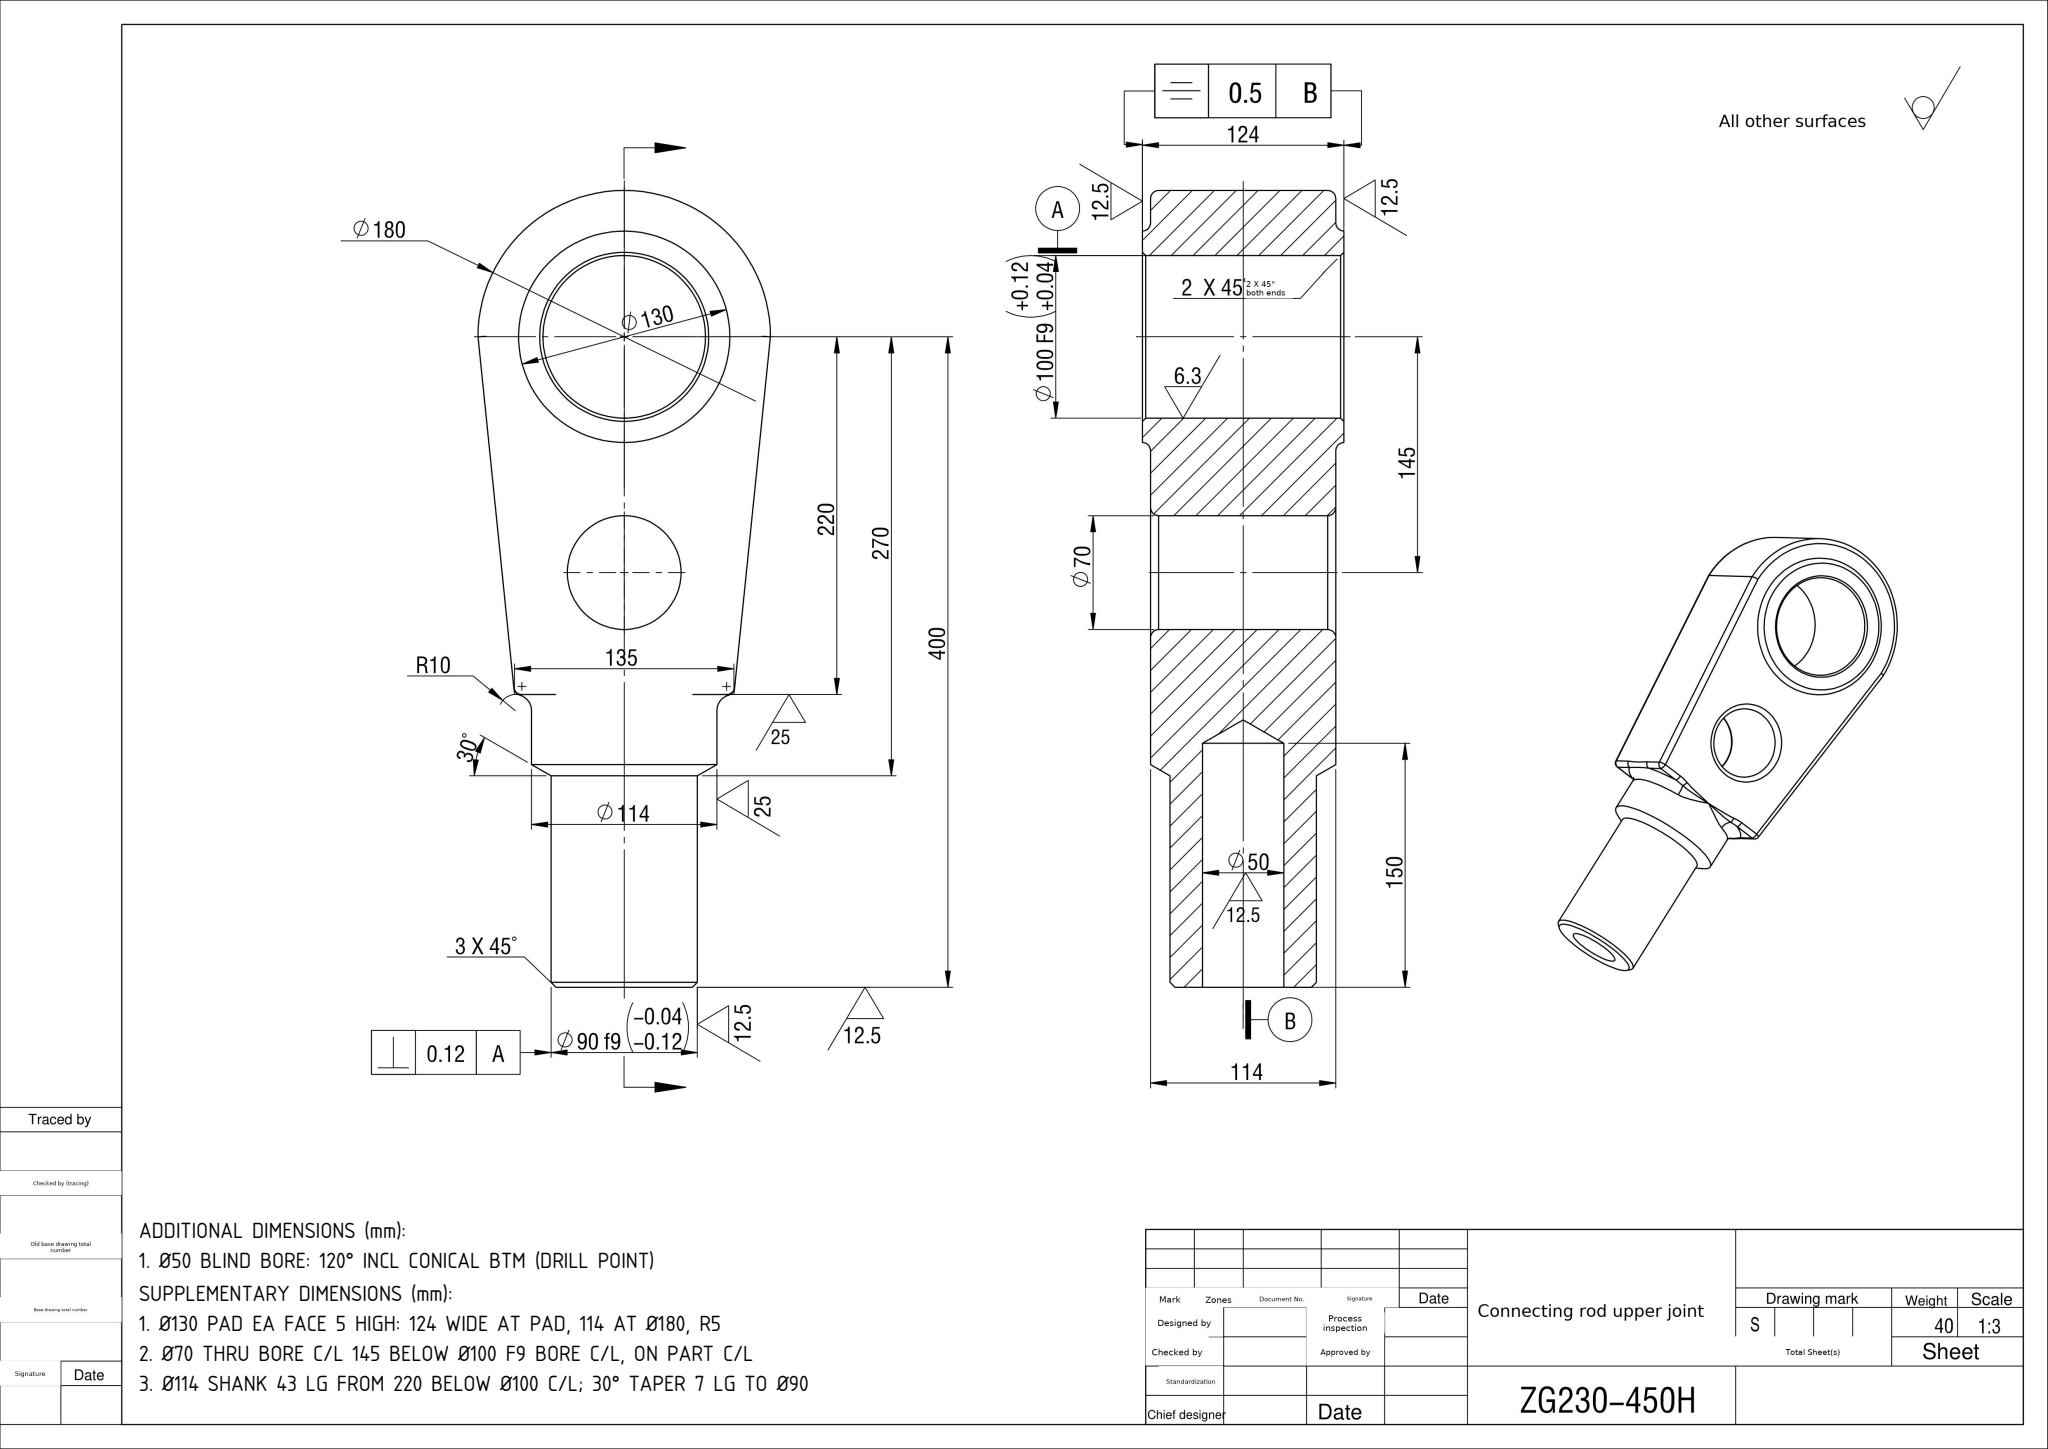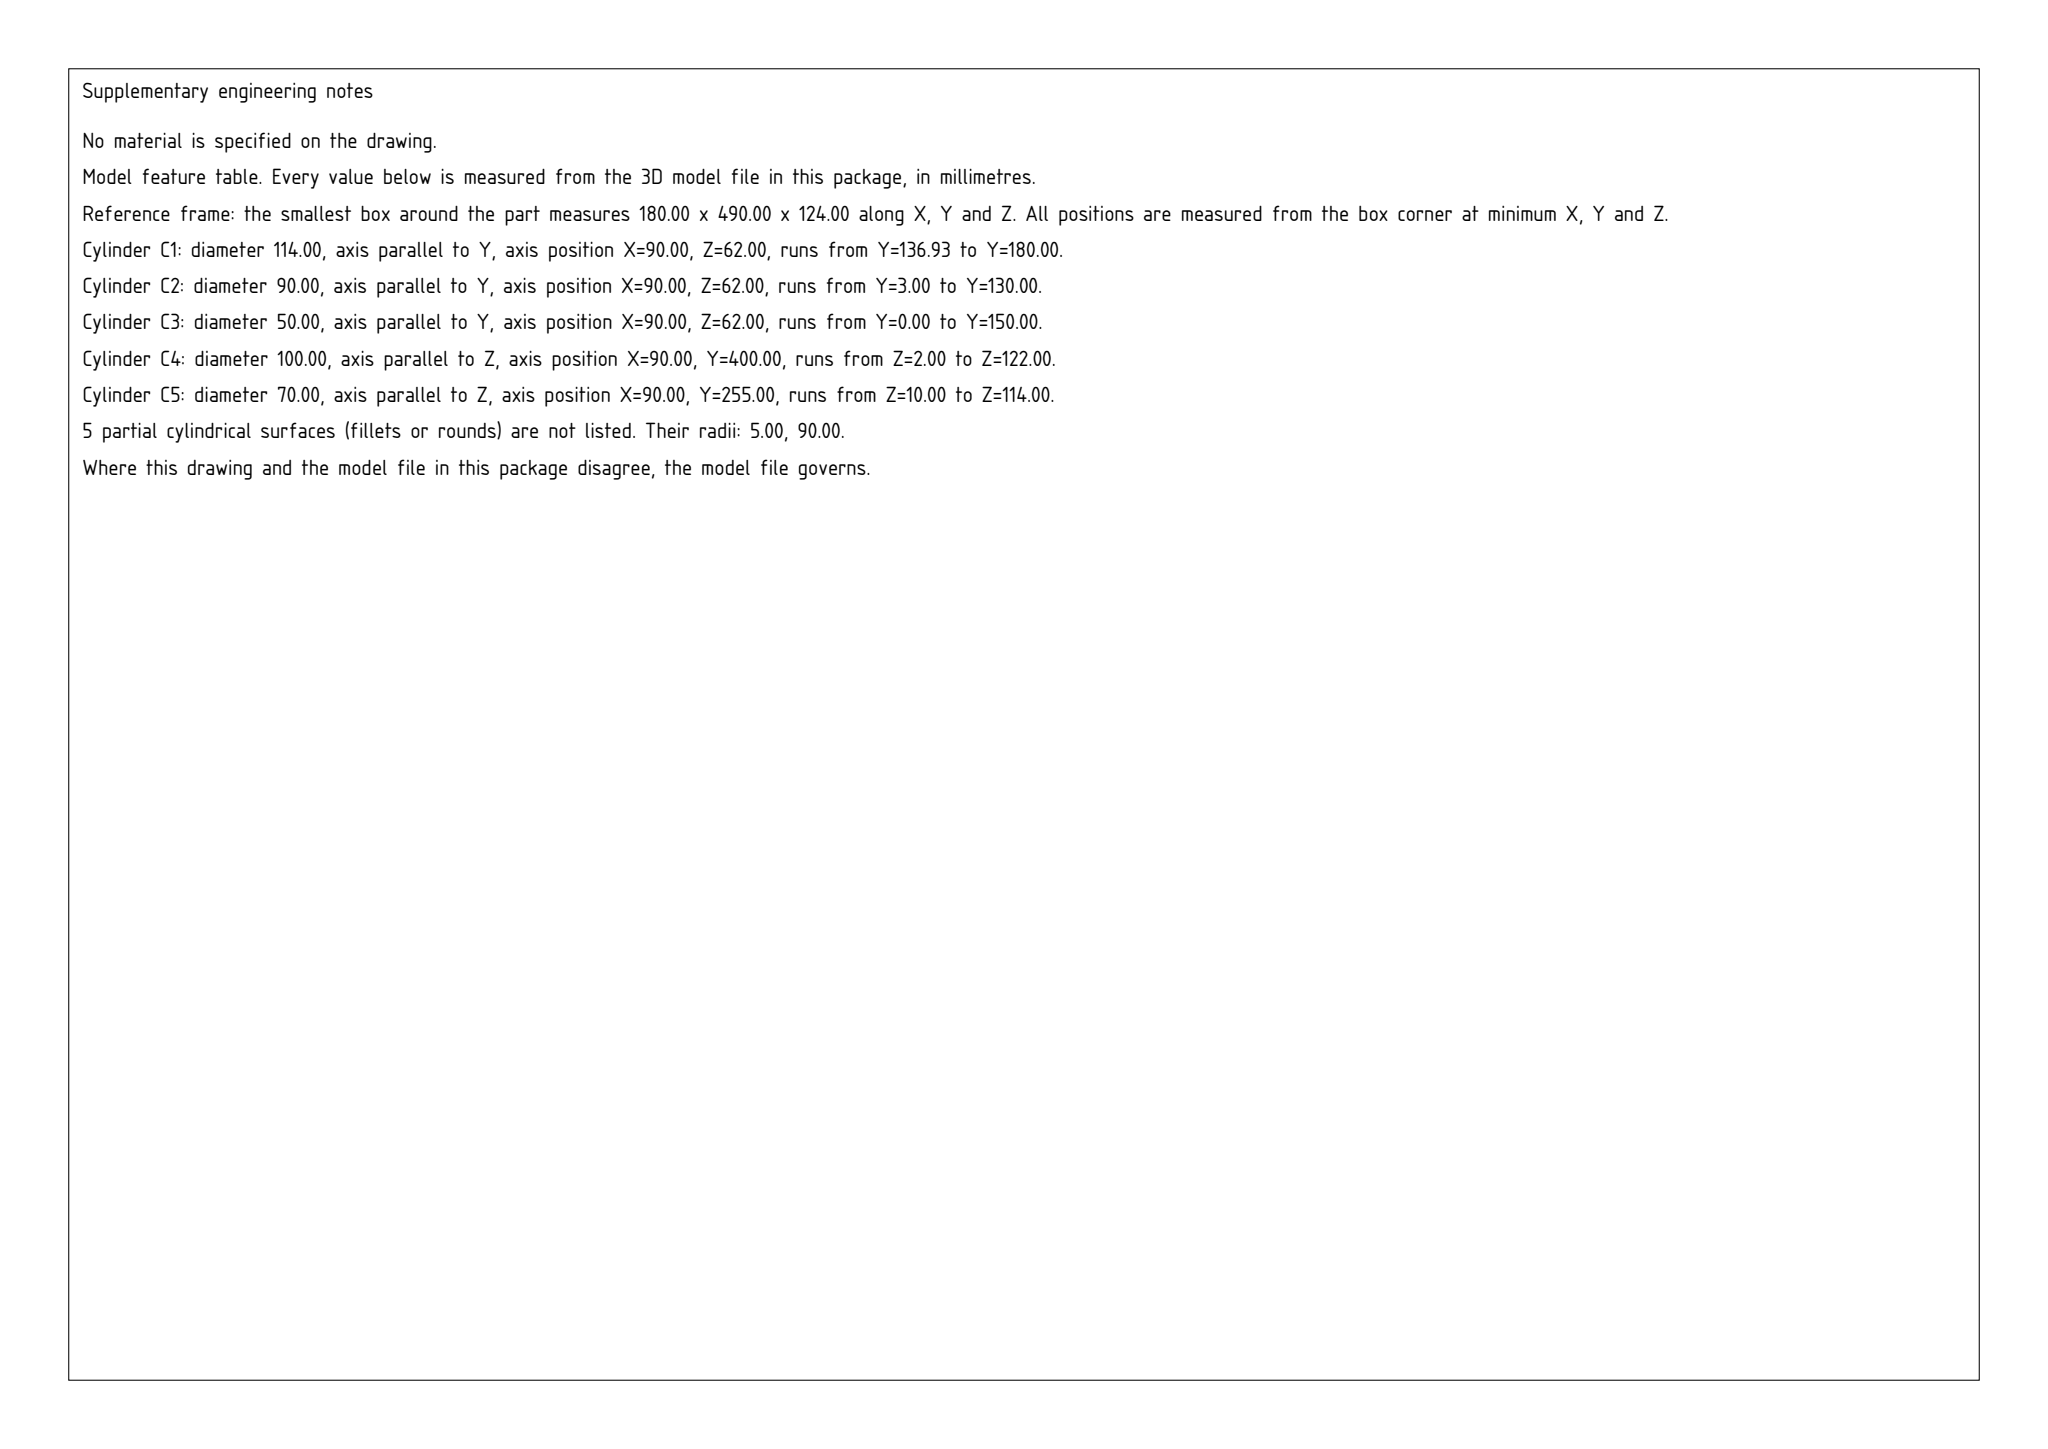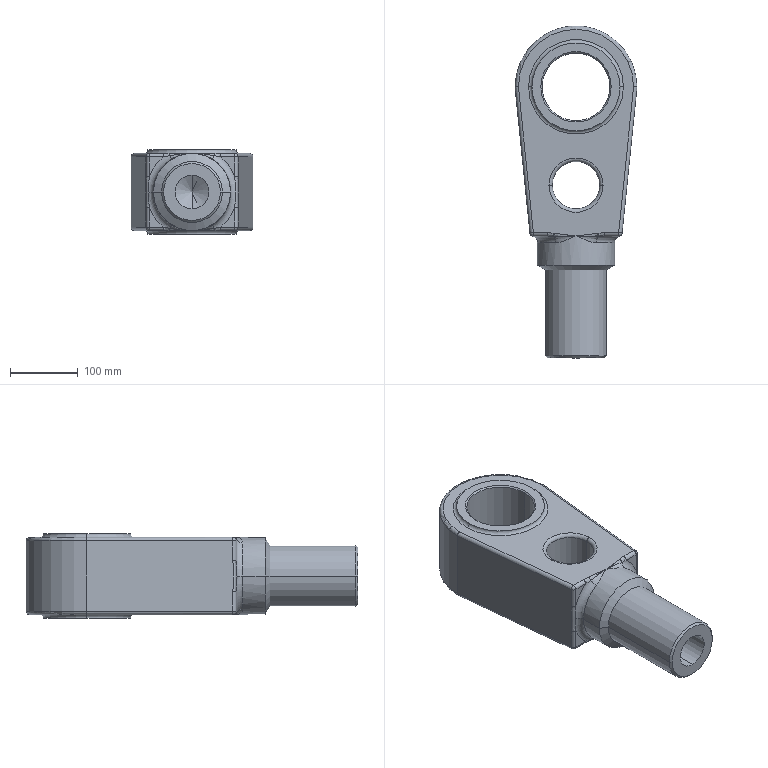Part | SolidWorks | mm | 1 solid | 75 faces | box 180 x 490 x 124 mm | volume 5136568 mm3 | cylinder 23 | spline 14 | torus 13 | plane 11 | cone 10 | sphere 4 | commonest cylinder face diameters 10 x12 50 x2 100 x2 90 x2 114 x2 70 x2 180 x1